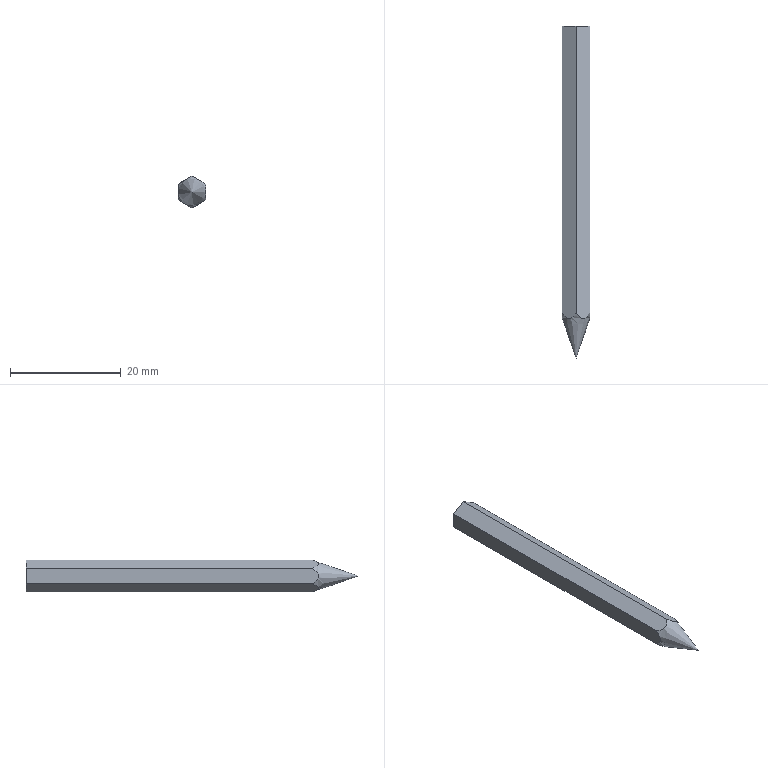Component | NX | 06 | 1 solid | 8 faces | box 5 x 60 x 5.77 mm | volume 1190 mm3 | plane 7 | cone 1
STEP:
#1=CARTESIAN_POINT('',(0.,0.,0.));
#2=DIRECTION('',(0.,0.,1.));
#3=DIRECTION('',(1.,0.,0.));
#4=AXIS2_PLACEMENT_3D('',#1,#2,#3);
#5=CARTESIAN_POINT('',(-22.043,-44.169,-1.443));
#6=VERTEX_POINT('',#5);
#7=CARTESIAN_POINT('',(-22.043,-95.922,-1.443));
#8=VERTEX_POINT('',#7);
#9=CARTESIAN_POINT('',(-22.043,-44.169,-1.443));
#10=DIRECTION('',(0.,-1.,0.));
#11=VECTOR('',#10,1.);
#12=LINE('',#9,#11);
#13=CARTESIAN_POINT('',(-22.043,-44.169,1.443));
#14=DIRECTION('',(-1.,0.,-0.));
#15=DIRECTION('',(0.,0.,-1.));
#16=AXIS2_PLACEMENT_3D('',#13,#14,#15);
#17=PLANE('',#16);
#18=CARTESIAN_POINT('',(2.887,0.));
#19=DIRECTION('',(0.,1.));
#20=VECTOR('',#19,1.);
#21=LINE('',#18,#20);
#22=(GEOMETRIC_REPRESENTATION_CONTEXT(2)PARAMETRIC_REPRESENTATION_CONTEXT()REPRESENTATION_CONTEXT('',''));
#23=DEFINITIONAL_REPRESENTATION('',(#21),#22);
#24=PCURVE('',#17,#23);
#25=CARTESIAN_POINT('',(-22.043,-44.169,-1.443));
#26=DIRECTION('',(-0.5,0.,-0.866));
#27=DIRECTION('',(0.866,0.,-0.5));
#28=AXIS2_PLACEMENT_3D('',#25,#26,#27);
#29=PLANE('',#28);
#30=CARTESIAN_POINT('',(0.,0.));
#31=DIRECTION('',(0.,1.));
#32=VECTOR('',#31,1.);
#33=LINE('',#30,#32);
#34=(GEOMETRIC_REPRESENTATION_CONTEXT(2)PARAMETRIC_REPRESENTATION_CONTEXT()REPRESENTATION_CONTEXT('',''));
#35=DEFINITIONAL_REPRESENTATION('',(#33),#34);
#36=PCURVE('',#29,#35);
#37=SURFACE_CURVE('',#12,(#24,#36),.PCURVE_S1.);
#38=EDGE_CURVE('',#6,#8,#37,.T.);
#39=ORIENTED_EDGE('',*,*,#38,.T.);
#40=CARTESIAN_POINT('',(-22.043,-95.922,1.443));
#41=VERTEX_POINT('',#40);
#42=CARTESIAN_POINT('',(-22.043,-95.922,1.443));
#43=CARTESIAN_POINT('',(-22.043,-96.22,1.235));
#44=CARTESIAN_POINT('',(-22.043,-96.512,1.004));
#45=CARTESIAN_POINT('',(-22.043,-96.738,0.7181));
#46=CARTESIAN_POINT('',(-22.043,-96.826,0.6057));
#47=CARTESIAN_POINT('',(-22.043,-96.905,0.4823));
#48=CARTESIAN_POINT('',(-22.043,-96.957,0.3493));
#49=CARTESIAN_POINT('',(-22.043,-96.996,0.2517));
#50=CARTESIAN_POINT('',(-22.043,-97.02,0.1468));
#51=CARTESIAN_POINT('',(-22.043,-97.026,0.04207));
#52=CARTESIAN_POINT('',(-22.043,-97.031,-0.06307));
#53=CARTESIAN_POINT('',(-22.043,-97.016,-0.1705));
#54=CARTESIAN_POINT('',(-22.043,-96.985,-0.2711));
#55=CARTESIAN_POINT('',(-22.043,-96.944,-0.4017));
#56=CARTESIAN_POINT('',(-22.043,-96.877,-0.5249));
#57=CARTESIAN_POINT('',(-22.043,-96.799,-0.6366));
#58=CARTESIAN_POINT('',(-22.043,-96.614,-0.8978));
#59=CARTESIAN_POINT('',(-22.043,-96.366,-1.113));
#60=CARTESIAN_POINT('',(-22.043,-96.111,-1.305));
#61=CARTESIAN_POINT('',(-22.043,-96.049,-1.353));
#62=CARTESIAN_POINT('',(-22.043,-95.986,-1.399));
#63=CARTESIAN_POINT('',(-22.043,-95.922,-1.443));
#64=B_SPLINE_CURVE_WITH_KNOTS('',3,(#42,#43,#44,#45,#46,#47,#48,#49,#50,#51,#52,#53,#54,#55,#56,#57,#58,#59,#60,#61,#62,#63),.UNSPECIFIED.,.F.,.F.,(4,3,3,3,3,3,3,4),(0.,0.2915,0.4053,0.4887,0.5725,0.6814,0.9377,1.),.UNSPECIFIED.);
#65=CARTESIAN_POINT('',(0.,51.752));
#66=CARTESIAN_POINT('',(0.2087,52.05));
#67=CARTESIAN_POINT('',(0.4395,52.343));
#68=CARTESIAN_POINT('',(0.7253,52.568));
#69=CARTESIAN_POINT('',(0.8376,52.657));
#70=CARTESIAN_POINT('',(0.9611,52.735));
#71=CARTESIAN_POINT('',(1.094,52.788));
#72=CARTESIAN_POINT('',(1.192,52.826));
#73=CARTESIAN_POINT('',(1.297,52.851));
#74=CARTESIAN_POINT('',(1.401,52.856));
#75=CARTESIAN_POINT('',(1.506,52.861));
#76=CARTESIAN_POINT('',(1.614,52.846));
#77=CARTESIAN_POINT('',(1.714,52.815));
#78=CARTESIAN_POINT('',(1.845,52.775));
#79=CARTESIAN_POINT('',(1.968,52.708));
#80=CARTESIAN_POINT('',(2.08,52.629));
#81=CARTESIAN_POINT('',(2.341,52.445));
#82=CARTESIAN_POINT('',(2.556,52.197));
#83=CARTESIAN_POINT('',(2.749,51.942));
#84=CARTESIAN_POINT('',(2.796,51.88));
#85=CARTESIAN_POINT('',(2.842,51.816));
#86=CARTESIAN_POINT('',(2.887,51.752));
#87=B_SPLINE_CURVE_WITH_KNOTS('',3,(#65,#66,#67,#68,#69,#70,#71,#72,#73,#74,#75,#76,#77,#78,#79,#80,#81,#82,#83,#84,#85,#86),.UNSPECIFIED.,.F.,.F.,(4,3,3,3,3,3,3,4),(0.,0.2915,0.4053,0.4887,0.5725,0.6814,0.9377,1.),.UNSPECIFIED.);
#88=(GEOMETRIC_REPRESENTATION_CONTEXT(2)PARAMETRIC_REPRESENTATION_CONTEXT()REPRESENTATION_CONTEXT('',''));
#89=DEFINITIONAL_REPRESENTATION('',(#87),#88);
#90=PCURVE('',#17,#89);
#91=CARTESIAN_POINT('',(-19.543,-104.169,0.00000003));
#92=DIRECTION('',(0.,1.,0.));
#93=DIRECTION('',(0.866,0.,-0.5));
#94=AXIS2_PLACEMENT_3D('',#91,#92,#93);
#95=CONICAL_SURFACE('',#94,0.,0.3367);
#96=CARTESIAN_POINT('',(3.142,8.248));
#97=CARTESIAN_POINT('',(3.137,8.225));
#98=CARTESIAN_POINT('',(3.127,8.178));
#99=CARTESIAN_POINT('',(3.111,8.109));
#100=CARTESIAN_POINT('',(3.095,8.04));
#101=CARTESIAN_POINT('',(3.079,7.972));
#102=CARTESIAN_POINT('',(3.061,7.905));
#103=CARTESIAN_POINT('',(3.044,7.839));
#104=CARTESIAN_POINT('',(3.025,7.775));
#105=CARTESIAN_POINT('',(3.005,7.711));
#106=CARTESIAN_POINT('',(2.985,7.65));
#107=CARTESIAN_POINT('',(2.963,7.59));
#108=CARTESIAN_POINT('',(2.941,7.532));
#109=CARTESIAN_POINT('',(2.918,7.476));
#110=CARTESIAN_POINT('',(2.894,7.422));
#111=CARTESIAN_POINT('',(2.868,7.371));
#112=CARTESIAN_POINT('',(2.841,7.323));
#113=CARTESIAN_POINT('',(2.812,7.279));
#114=CARTESIAN_POINT('',(2.783,7.24));
#115=CARTESIAN_POINT('',(2.752,7.206));
#116=CARTESIAN_POINT('',(2.72,7.179));
#117=CARTESIAN_POINT('',(2.686,7.158));
#118=CARTESIAN_POINT('',(2.652,7.146));
#119=CARTESIAN_POINT('',(2.618,7.141));
#120=CARTESIAN_POINT('',(2.583,7.146));
#121=CARTESIAN_POINT('',(2.549,7.159));
#122=CARTESIAN_POINT('',(2.516,7.179));
#123=CARTESIAN_POINT('',(2.484,7.206));
#124=CARTESIAN_POINT('',(2.453,7.24));
#125=CARTESIAN_POINT('',(2.423,7.279));
#126=CARTESIAN_POINT('',(2.395,7.323));
#127=CARTESIAN_POINT('',(2.368,7.371));
#128=CARTESIAN_POINT('',(2.343,7.422));
#129=CARTESIAN_POINT('',(2.318,7.475));
#130=CARTESIAN_POINT('',(2.295,7.531));
#131=CARTESIAN_POINT('',(2.273,7.589));
#132=CARTESIAN_POINT('',(2.251,7.649));
#133=CARTESIAN_POINT('',(2.231,7.711));
#134=CARTESIAN_POINT('',(2.211,7.775));
#135=CARTESIAN_POINT('',(2.193,7.84));
#136=CARTESIAN_POINT('',(2.175,7.906));
#137=CARTESIAN_POINT('',(2.157,7.973));
#138=CARTESIAN_POINT('',(2.141,8.04));
#139=CARTESIAN_POINT('',(2.125,8.109));
#140=CARTESIAN_POINT('',(2.109,8.178));
#141=CARTESIAN_POINT('',(2.099,8.224));
#142=CARTESIAN_POINT('',(2.094,8.248));
#143=B_SPLINE_CURVE_WITH_KNOTS('',3,(#96,#97,#98,#99,#100,#101,#102,#103,#104,#105,#106,#107,#108,#109,#110,#111,#112,#113,#114,#115,#116,#117,#118,#119,#120,#121,#122,#123,#124,#125,#126,#127,#128,#129,#130,#131,#132,#133,#134,#135,#136,#137,#138,#139,#140,#141,#142),.UNSPECIFIED.,.F.,.F.,(4,1,1,1,1,1,1,1,1,1,1,1,1,1,1,1,1,1,1,1,1,1,1,1,1,1,1,1,1,1,1,1,1,1,1,1,1,1,1,1,1,1,1,1,4),(0.,0.02273,0.04545,0.06818,0.09091,0.1136,0.1364,0.1591,0.1818,0.2045,0.2273,0.25,0.2727,0.2955,0.3182,0.3409,0.3636,0.3864,0.4091,0.4318,0.4545,0.4773,0.5,0.5227,0.5455,0.5682,0.5909,0.6136,0.6364,0.6591,0.6818,0.7045,0.7273,0.75,0.7727,0.7955,0.8182,0.8409,0.8636,0.8864,0.9091,0.9318,0.9545,0.9773,1.),.QUASI_UNIFORM_KNOTS.);
#144=(GEOMETRIC_REPRESENTATION_CONTEXT(2)PARAMETRIC_REPRESENTATION_CONTEXT()REPRESENTATION_CONTEXT('',''));
#145=DEFINITIONAL_REPRESENTATION('',(#143),#144);
#146=PCURVE('',#95,#145);
#147=SURFACE_CURVE('',#64,(#90,#146),.PCURVE_S1.);
#148=EDGE_CURVE('',#41,#8,#147,.T.);
#149=ORIENTED_EDGE('',*,*,#148,.F.);
#150=CARTESIAN_POINT('',(-22.043,-44.169,1.443));
#151=VERTEX_POINT('',#150);
#152=CARTESIAN_POINT('',(-22.043,-44.169,1.443));
#153=DIRECTION('',(0.,-1.,0.));
#154=VECTOR('',#153,1.);
#155=LINE('',#152,#154);
#156=CARTESIAN_POINT('',(0.,0.));
#157=DIRECTION('',(0.,1.));
#158=VECTOR('',#157,1.);
#159=LINE('',#156,#158);
#160=(GEOMETRIC_REPRESENTATION_CONTEXT(2)PARAMETRIC_REPRESENTATION_CONTEXT()REPRESENTATION_CONTEXT('',''));
#161=DEFINITIONAL_REPRESENTATION('',(#159),#160);
#162=PCURVE('',#17,#161);
#163=CARTESIAN_POINT('',(-19.543,-44.169,2.887));
#164=DIRECTION('',(-0.5,0.,0.866));
#165=DIRECTION('',(-0.866,0.,-0.5));
#166=AXIS2_PLACEMENT_3D('',#163,#164,#165);
#167=PLANE('',#166);
#168=CARTESIAN_POINT('',(2.887,0.));
#169=DIRECTION('',(0.,1.));
#170=VECTOR('',#169,1.);
#171=LINE('',#168,#170);
#172=(GEOMETRIC_REPRESENTATION_CONTEXT(2)PARAMETRIC_REPRESENTATION_CONTEXT()REPRESENTATION_CONTEXT('',''));
#173=DEFINITIONAL_REPRESENTATION('',(#171),#172);
#174=PCURVE('',#167,#173);
#175=SURFACE_CURVE('',#155,(#162,#174),.PCURVE_S1.);
#176=EDGE_CURVE('',#151,#41,#175,.T.);
#177=ORIENTED_EDGE('',*,*,#176,.F.);
#178=CARTESIAN_POINT('',(-22.043,-44.169,1.443));
#179=DIRECTION('',(0.,0.,-1.));
#180=VECTOR('',#179,1.);
#181=LINE('',#178,#180);
#182=CARTESIAN_POINT('',(0.,0.));
#183=DIRECTION('',(1.,0.));
#184=VECTOR('',#183,1.);
#185=LINE('',#182,#184);
#186=(GEOMETRIC_REPRESENTATION_CONTEXT(2)PARAMETRIC_REPRESENTATION_CONTEXT()REPRESENTATION_CONTEXT('',''));
#187=DEFINITIONAL_REPRESENTATION('',(#185),#186);
#188=PCURVE('',#17,#187);
#189=CARTESIAN_POINT('',(-19.543,-44.169,0.00000003));
#190=DIRECTION('',(0.,-1.,0.));
#191=DIRECTION('',(0.866,0.,-0.5));
#192=AXIS2_PLACEMENT_3D('',#189,#190,#191);
#193=PLANE('',#192);
#194=CARTESIAN_POINT('',(-2.887,0.));
#195=DIRECTION('',(0.5,-0.866));
#196=VECTOR('',#195,1.);
#197=LINE('',#194,#196);
#198=(GEOMETRIC_REPRESENTATION_CONTEXT(2)PARAMETRIC_REPRESENTATION_CONTEXT()REPRESENTATION_CONTEXT('',''));
#199=DEFINITIONAL_REPRESENTATION('',(#197),#198);
#200=PCURVE('',#193,#199);
#201=SURFACE_CURVE('',#181,(#188,#200),.PCURVE_S1.);
#202=EDGE_CURVE('',#151,#6,#201,.T.);
#203=ORIENTED_EDGE('',*,*,#202,.T.);
#204=EDGE_LOOP('',(#39,#149,#177,#203));
#205=FACE_BOUND('',#204,.T.);
#206=ADVANCED_FACE('',(#205),#17,.T.);
#207=CARTESIAN_POINT('',(-19.543,-44.169,-2.887));
#208=VERTEX_POINT('',#207);
#209=CARTESIAN_POINT('',(-19.543,-95.922,-2.887));
#210=VERTEX_POINT('',#209);
#211=CARTESIAN_POINT('',(-19.543,-44.169,-2.887));
#212=DIRECTION('',(0.,-1.,0.));
#213=VECTOR('',#212,1.);
#214=LINE('',#211,#213);
#215=CARTESIAN_POINT('',(2.887,0.));
#216=DIRECTION('',(0.,1.));
#217=VECTOR('',#216,1.);
#218=LINE('',#215,#217);
#219=(GEOMETRIC_REPRESENTATION_CONTEXT(2)PARAMETRIC_REPRESENTATION_CONTEXT()REPRESENTATION_CONTEXT('',''));
#220=DEFINITIONAL_REPRESENTATION('',(#218),#219);
#221=PCURVE('',#29,#220);
#222=CARTESIAN_POINT('',(-19.543,-44.169,-2.887));
#223=DIRECTION('',(0.5,0.,-0.866));
#224=DIRECTION('',(0.866,0.,0.5));
#225=AXIS2_PLACEMENT_3D('',#222,#223,#224);
#226=PLANE('',#225);
#227=CARTESIAN_POINT('',(0.,0.));
#228=DIRECTION('',(0.,1.));
#229=VECTOR('',#228,1.);
#230=LINE('',#227,#229);
#231=(GEOMETRIC_REPRESENTATION_CONTEXT(2)PARAMETRIC_REPRESENTATION_CONTEXT()REPRESENTATION_CONTEXT('',''));
#232=DEFINITIONAL_REPRESENTATION('',(#230),#231);
#233=PCURVE('',#226,#232);
#234=SURFACE_CURVE('',#214,(#221,#233),.PCURVE_S1.);
#235=EDGE_CURVE('',#208,#210,#234,.T.);
#236=ORIENTED_EDGE('',*,*,#235,.T.);
#237=CARTESIAN_POINT('',(-22.043,-95.922,-1.443));
#238=CARTESIAN_POINT('',(-21.889,-96.175,-1.532));
#239=CARTESIAN_POINT('',(-21.72,-96.425,-1.63));
#240=CARTESIAN_POINT('',(-21.316,-96.848,-1.863));
#241=CARTESIAN_POINT('',(-21.066,-97.027,-2.007));
#242=CARTESIAN_POINT('',(-20.516,-97.026,-2.325));
#243=CARTESIAN_POINT('',(-20.267,-96.846,-2.469));
#244=CARTESIAN_POINT('',(-19.865,-96.424,-2.701));
#245=CARTESIAN_POINT('',(-19.698,-96.178,-2.797));
#246=CARTESIAN_POINT('',(-19.543,-95.922,-2.887));
#247=B_SPLINE_CURVE_WITH_KNOTS('',3,(#237,#238,#239,#240,#241,#242,#243,#244,#245,#246),.UNSPECIFIED.,.F.,.F.,(4,2,2,2,4),(0.,0.25,0.5,0.75,1.),.UNSPECIFIED.);
#248=CARTESIAN_POINT('',(0.,51.752));
#249=CARTESIAN_POINT('',(0.1777,52.006));
#250=CARTESIAN_POINT('',(0.3732,52.256));
#251=CARTESIAN_POINT('',(0.8395,52.679));
#252=CARTESIAN_POINT('',(1.128,52.858));
#253=CARTESIAN_POINT('',(1.763,52.857));
#254=CARTESIAN_POINT('',(2.051,52.676));
#255=CARTESIAN_POINT('',(2.515,52.254));
#256=CARTESIAN_POINT('',(2.707,52.009));
#257=CARTESIAN_POINT('',(2.887,51.752));
#258=B_SPLINE_CURVE_WITH_KNOTS('',3,(#248,#249,#250,#251,#252,#253,#254,#255,#256,#257),.UNSPECIFIED.,.F.,.F.,(4,2,2,2,4),(0.,0.25,0.5,0.75,1.),.UNSPECIFIED.);
#259=(GEOMETRIC_REPRESENTATION_CONTEXT(2)PARAMETRIC_REPRESENTATION_CONTEXT()REPRESENTATION_CONTEXT('',''));
#260=DEFINITIONAL_REPRESENTATION('',(#258),#259);
#261=PCURVE('',#29,#260);
#262=CARTESIAN_POINT('',(2.094,8.248));
#263=CARTESIAN_POINT('',(2.085,8.202));
#264=CARTESIAN_POINT('',(2.065,8.11));
#265=CARTESIAN_POINT('',(2.032,7.974));
#266=CARTESIAN_POINT('',(1.997,7.841));
#267=CARTESIAN_POINT('',(1.959,7.713));
#268=CARTESIAN_POINT('',(1.917,7.59));
#269=CARTESIAN_POINT('',(1.871,7.474));
#270=CARTESIAN_POINT('',(1.82,7.367));
#271=CARTESIAN_POINT('',(1.764,7.275));
#272=CARTESIAN_POINT('',(1.703,7.202));
#273=CARTESIAN_POINT('',(1.639,7.154));
#274=CARTESIAN_POINT('',(1.57,7.137));
#275=CARTESIAN_POINT('',(1.502,7.155));
#276=CARTESIAN_POINT('',(1.437,7.203));
#277=CARTESIAN_POINT('',(1.376,7.277));
#278=CARTESIAN_POINT('',(1.32,7.37));
#279=CARTESIAN_POINT('',(1.269,7.477));
#280=CARTESIAN_POINT('',(1.224,7.592));
#281=CARTESIAN_POINT('',(1.183,7.714));
#282=CARTESIAN_POINT('',(1.145,7.841));
#283=CARTESIAN_POINT('',(1.11,7.973));
#284=CARTESIAN_POINT('',(1.077,8.109));
#285=CARTESIAN_POINT('',(1.057,8.201));
#286=CARTESIAN_POINT('',(1.047,8.248));
#287=B_SPLINE_CURVE_WITH_KNOTS('',3,(#262,#263,#264,#265,#266,#267,#268,#269,#270,#271,#272,#273,#274,#275,#276,#277,#278,#279,#280,#281,#282,#283,#284,#285,#286),.UNSPECIFIED.,.F.,.F.,(4,1,1,1,1,1,1,1,1,1,1,1,1,1,1,1,1,1,1,1,1,1,4),(0.,0.04545,0.09091,0.1364,0.1818,0.2273,0.2727,0.3182,0.3636,0.4091,0.4545,0.5,0.5455,0.5909,0.6364,0.6818,0.7273,0.7727,0.8182,0.8636,0.9091,0.9545,1.),.QUASI_UNIFORM_KNOTS.);
#288=(GEOMETRIC_REPRESENTATION_CONTEXT(2)PARAMETRIC_REPRESENTATION_CONTEXT()REPRESENTATION_CONTEXT('',''));
#289=DEFINITIONAL_REPRESENTATION('',(#287),#288);
#290=PCURVE('',#95,#289);
#291=SURFACE_CURVE('',#247,(#261,#290),.PCURVE_S1.);
#292=EDGE_CURVE('',#8,#210,#291,.T.);
#293=ORIENTED_EDGE('',*,*,#292,.F.);
#294=ORIENTED_EDGE('',*,*,#38,.F.);
#295=CARTESIAN_POINT('',(-22.043,-44.169,-1.443));
#296=DIRECTION('',(0.866,0.,-0.5));
#297=VECTOR('',#296,1.);
#298=LINE('',#295,#297);
#299=CARTESIAN_POINT('',(0.,0.));
#300=DIRECTION('',(1.,0.));
#301=VECTOR('',#300,1.);
#302=LINE('',#299,#301);
#303=(GEOMETRIC_REPRESENTATION_CONTEXT(2)PARAMETRIC_REPRESENTATION_CONTEXT()REPRESENTATION_CONTEXT('',''));
#304=DEFINITIONAL_REPRESENTATION('',(#302),#303);
#305=PCURVE('',#29,#304);
#306=CARTESIAN_POINT('',(-1.443,-2.5));
#307=DIRECTION('',(1.,0.));
#308=VECTOR('',#307,1.);
#309=LINE('',#306,#308);
#310=(GEOMETRIC_REPRESENTATION_CONTEXT(2)PARAMETRIC_REPRESENTATION_CONTEXT()REPRESENTATION_CONTEXT('',''));
#311=DEFINITIONAL_REPRESENTATION('',(#309),#310);
#312=PCURVE('',#193,#311);
#313=SURFACE_CURVE('',#298,(#305,#312),.PCURVE_S1.);
#314=EDGE_CURVE('',#6,#208,#313,.T.);
#315=ORIENTED_EDGE('',*,*,#314,.T.);
#316=EDGE_LOOP('',(#236,#293,#294,#315));
#317=FACE_BOUND('',#316,.T.);
#318=ADVANCED_FACE('',(#317),#29,.T.);
#319=CARTESIAN_POINT('',(-17.043,-44.169,-1.443));
#320=VERTEX_POINT('',#319);
#321=CARTESIAN_POINT('',(-17.043,-95.922,-1.443));
#322=VERTEX_POINT('',#321);
#323=CARTESIAN_POINT('',(-17.043,-44.169,-1.443));
#324=DIRECTION('',(0.,-1.,0.));
#325=VECTOR('',#324,1.);
#326=LINE('',#323,#325);
#327=CARTESIAN_POINT('',(2.887,0.));
#328=DIRECTION('',(0.,1.));
#329=VECTOR('',#328,1.);
#330=LINE('',#327,#329);
#331=(GEOMETRIC_REPRESENTATION_CONTEXT(2)PARAMETRIC_REPRESENTATION_CONTEXT()REPRESENTATION_CONTEXT('',''));
#332=DEFINITIONAL_REPRESENTATION('',(#330),#331);
#333=PCURVE('',#226,#332);
#334=CARTESIAN_POINT('',(-17.043,-44.169,-1.443));
#335=DIRECTION('',(1.,0.,0.));
#336=DIRECTION('',(-0.,0.,1.));
#337=AXIS2_PLACEMENT_3D('',#334,#335,#336);
#338=PLANE('',#337);
#339=CARTESIAN_POINT('',(0.,0.));
#340=DIRECTION('',(0.,1.));
#341=VECTOR('',#340,1.);
#342=LINE('',#339,#341);
#343=(GEOMETRIC_REPRESENTATION_CONTEXT(2)PARAMETRIC_REPRESENTATION_CONTEXT()REPRESENTATION_CONTEXT('',''));
#344=DEFINITIONAL_REPRESENTATION('',(#342),#343);
#345=PCURVE('',#338,#344);
#346=SURFACE_CURVE('',#326,(#333,#345),.PCURVE_S1.);
#347=EDGE_CURVE('',#320,#322,#346,.T.);
#348=ORIENTED_EDGE('',*,*,#347,.T.);
#349=CARTESIAN_POINT('',(-19.543,-95.922,-2.887));
#350=CARTESIAN_POINT('',(-19.362,-96.22,-2.782));
#351=CARTESIAN_POINT('',(-19.162,-96.512,-2.667));
#352=CARTESIAN_POINT('',(-18.915,-96.738,-2.524));
#353=CARTESIAN_POINT('',(-18.817,-96.826,-2.468));
#354=CARTESIAN_POINT('',(-18.711,-96.905,-2.406));
#355=CARTESIAN_POINT('',(-18.595,-96.957,-2.34));
#356=CARTESIAN_POINT('',(-18.511,-96.996,-2.291));
#357=CARTESIAN_POINT('',(-18.42,-97.02,-2.238));
#358=CARTESIAN_POINT('',(-18.329,-97.026,-2.186));
#359=CARTESIAN_POINT('',(-18.238,-97.031,-2.134));
#360=CARTESIAN_POINT('',(-18.145,-97.016,-2.08));
#361=CARTESIAN_POINT('',(-18.058,-96.985,-2.03));
#362=CARTESIAN_POINT('',(-17.945,-96.944,-1.964));
#363=CARTESIAN_POINT('',(-17.838,-96.877,-1.903));
#364=CARTESIAN_POINT('',(-17.742,-96.799,-1.847));
#365=CARTESIAN_POINT('',(-17.515,-96.614,-1.716));
#366=CARTESIAN_POINT('',(-17.329,-96.366,-1.609));
#367=CARTESIAN_POINT('',(-17.162,-96.111,-1.512));
#368=CARTESIAN_POINT('',(-17.121,-96.049,-1.489));
#369=CARTESIAN_POINT('',(-17.082,-95.986,-1.466));
#370=CARTESIAN_POINT('',(-17.043,-95.922,-1.443));
#371=B_SPLINE_CURVE_WITH_KNOTS('',3,(#349,#350,#351,#352,#353,#354,#355,#356,#357,#358,#359,#360,#361,#362,#363,#364,#365,#366,#367,#368,#369,#370),.UNSPECIFIED.,.F.,.F.,(4,3,3,3,3,3,3,4),(0.,0.2915,0.4053,0.4887,0.5725,0.6814,0.9377,1.),.UNSPECIFIED.);
#372=CARTESIAN_POINT('',(0.,51.752));
#373=CARTESIAN_POINT('',(0.2087,52.05));
#374=CARTESIAN_POINT('',(0.4395,52.343));
#375=CARTESIAN_POINT('',(0.7253,52.568));
#376=CARTESIAN_POINT('',(0.8376,52.657));
#377=CARTESIAN_POINT('',(0.9611,52.735));
#378=CARTESIAN_POINT('',(1.094,52.788));
#379=CARTESIAN_POINT('',(1.192,52.826));
#380=CARTESIAN_POINT('',(1.297,52.851));
#381=CARTESIAN_POINT('',(1.401,52.856));
#382=CARTESIAN_POINT('',(1.506,52.861));
#383=CARTESIAN_POINT('',(1.614,52.846));
#384=CARTESIAN_POINT('',(1.714,52.815));
#385=CARTESIAN_POINT('',(1.845,52.775));
#386=CARTESIAN_POINT('',(1.968,52.708));
#387=CARTESIAN_POINT('',(2.08,52.629));
#388=CARTESIAN_POINT('',(2.341,52.445));
#389=CARTESIAN_POINT('',(2.556,52.197));
#390=CARTESIAN_POINT('',(2.749,51.942));
#391=CARTESIAN_POINT('',(2.796,51.88));
#392=CARTESIAN_POINT('',(2.842,51.816));
#393=CARTESIAN_POINT('',(2.887,51.752));
#394=B_SPLINE_CURVE_WITH_KNOTS('',3,(#372,#373,#374,#375,#376,#377,#378,#379,#380,#381,#382,#383,#384,#385,#386,#387,#388,#389,#390,#391,#392,#393),.UNSPECIFIED.,.F.,.F.,(4,3,3,3,3,3,3,4),(0.,0.2915,0.4053,0.4887,0.5725,0.6814,0.9377,1.),.UNSPECIFIED.);
#395=(GEOMETRIC_REPRESENTATION_CONTEXT(2)PARAMETRIC_REPRESENTATION_CONTEXT()REPRESENTATION_CONTEXT('',''));
#396=DEFINITIONAL_REPRESENTATION('',(#394),#395);
#397=PCURVE('',#226,#396);
#398=CARTESIAN_POINT('',(1.047,8.248));
#399=CARTESIAN_POINT('',(1.042,8.225));
#400=CARTESIAN_POINT('',(1.032,8.178));
#401=CARTESIAN_POINT('',(1.017,8.109));
#402=CARTESIAN_POINT('',(1.001,8.04));
#403=CARTESIAN_POINT('',(0.9844,7.972));
#404=CARTESIAN_POINT('',(0.9671,7.905));
#405=CARTESIAN_POINT('',(0.9491,7.839));
#406=CARTESIAN_POINT('',(0.9304,7.775));
#407=CARTESIAN_POINT('',(0.9108,7.711));
#408=CARTESIAN_POINT('',(0.8904,7.65));
#409=CARTESIAN_POINT('',(0.8691,7.59));
#410=CARTESIAN_POINT('',(0.8468,7.532));
#411=CARTESIAN_POINT('',(0.8235,7.476));
#412=CARTESIAN_POINT('',(0.7992,7.422));
#413=CARTESIAN_POINT('',(0.7734,7.371));
#414=CARTESIAN_POINT('',(0.7464,7.323));
#415=CARTESIAN_POINT('',(0.718,7.279));
#416=CARTESIAN_POINT('',(0.6883,7.24));
#417=CARTESIAN_POINT('',(0.6574,7.206));
#418=CARTESIAN_POINT('',(0.6252,7.179));
#419=CARTESIAN_POINT('',(0.5918,7.158));
#420=CARTESIAN_POINT('',(0.5577,7.146));
#421=CARTESIAN_POINT('',(0.5234,7.141));
#422=CARTESIAN_POINT('',(0.489,7.146));
#423=CARTESIAN_POINT('',(0.4549,7.159));
#424=CARTESIAN_POINT('',(0.4216,7.179));
#425=CARTESIAN_POINT('',(0.3896,7.206));
#426=CARTESIAN_POINT('',(0.3586,7.24));
#427=CARTESIAN_POINT('',(0.3289,7.279));
#428=CARTESIAN_POINT('',(0.3005,7.323));
#429=CARTESIAN_POINT('',(0.2735,7.371));
#430=CARTESIAN_POINT('',(0.2481,7.422));
#431=CARTESIAN_POINT('',(0.2237,7.475));
#432=CARTESIAN_POINT('',(0.2004,7.531));
#433=CARTESIAN_POINT('',(0.1782,7.589));
#434=CARTESIAN_POINT('',(0.1569,7.649));
#435=CARTESIAN_POINT('',(0.1365,7.711));
#436=CARTESIAN_POINT('',(0.117,7.775));
#437=CARTESIAN_POINT('',(0.09826,7.84));
#438=CARTESIAN_POINT('',(0.08031,7.906));
#439=CARTESIAN_POINT('',(0.06307,7.973));
#440=CARTESIAN_POINT('',(0.04652,8.04));
#441=CARTESIAN_POINT('',(0.03043,8.109));
#442=CARTESIAN_POINT('',(0.01491,8.178));
#443=CARTESIAN_POINT('',(0.004909,8.224));
#444=CARTESIAN_POINT('',(0.,8.248));
#445=B_SPLINE_CURVE_WITH_KNOTS('',3,(#398,#399,#400,#401,#402,#403,#404,#405,#406,#407,#408,#409,#410,#411,#412,#413,#414,#415,#416,#417,#418,#419,#420,#421,#422,#423,#424,#425,#426,#427,#428,#429,#430,#431,#432,#433,#434,#435,#436,#437,#438,#439,#440,#441,#442,#443,#444),.UNSPECIFIED.,.F.,.F.,(4,1,1,1,1,1,1,1,1,1,1,1,1,1,1,1,1,1,1,1,1,1,1,1,1,1,1,1,1,1,1,1,1,1,1,1,1,1,1,1,1,1,1,1,4),(0.,0.02273,0.04545,0.06818,0.09091,0.1136,0.1364,0.1591,0.1818,0.2045,0.2273,0.25,0.2727,0.2955,0.3182,0.3409,0.3636,0.3864,0.4091,0.4318,0.4545,0.4773,0.5,0.5227,0.5455,0.5682,0.5909,0.6136,0.6364,0.6591,0.6818,0.7045,0.7273,0.75,0.7727,0.7955,0.8182,0.8409,0.8636,0.8864,0.9091,0.9318,0.9545,0.9773,1.),.QUASI_UNIFORM_KNOTS.);
#446=(GEOMETRIC_REPRESENTATION_CONTEXT(2)PARAMETRIC_REPRESENTATION_CONTEXT()REPRESENTATION_CONTEXT('',''));
#447=DEFINITIONAL_REPRESENTATION('',(#445),#446);
#448=PCURVE('',#95,#447);
#449=SURFACE_CURVE('',#371,(#397,#448),.PCURVE_S1.);
#450=EDGE_CURVE('',#210,#322,#449,.T.);
#451=ORIENTED_EDGE('',*,*,#450,.F.);
#452=ORIENTED_EDGE('',*,*,#235,.F.);
#453=CARTESIAN_POINT('',(-19.543,-44.169,-2.887));
#454=DIRECTION('',(0.866,0.,0.5));
#455=VECTOR('',#454,1.);
#456=LINE('',#453,#455);
#457=CARTESIAN_POINT('',(0.,0.));
#458=DIRECTION('',(1.,0.));
#459=VECTOR('',#458,1.);
#460=LINE('',#457,#459);
#461=(GEOMETRIC_REPRESENTATION_CONTEXT(2)PARAMETRIC_REPRESENTATION_CONTEXT()REPRESENTATION_CONTEXT('',''));
#462=DEFINITIONAL_REPRESENTATION('',(#460),#461);
#463=PCURVE('',#226,#462);
#464=CARTESIAN_POINT('',(1.443,-2.5));
#465=DIRECTION('',(0.5,0.866));
#466=VECTOR('',#465,1.);
#467=LINE('',#464,#466);
#468=(GEOMETRIC_REPRESENTATION_CONTEXT(2)PARAMETRIC_REPRESENTATION_CONTEXT()REPRESENTATION_CONTEXT('',''));
#469=DEFINITIONAL_REPRESENTATION('',(#467),#468);
#470=PCURVE('',#193,#469);
#471=SURFACE_CURVE('',#456,(#463,#470),.PCURVE_S1.);
#472=EDGE_CURVE('',#208,#320,#471,.T.);
#473=ORIENTED_EDGE('',*,*,#472,.T.);
#474=EDGE_LOOP('',(#348,#451,#452,#473));
#475=FACE_BOUND('',#474,.T.);
#476=ADVANCED_FACE('',(#475),#226,.T.);
#477=CARTESIAN_POINT('',(-17.043,-44.169,1.443));
#478=VERTEX_POINT('',#477);
#479=CARTESIAN_POINT('',(-17.043,-95.922,1.443));
#480=VERTEX_POINT('',#479);
#481=CARTESIAN_POINT('',(-17.043,-44.169,1.443));
#482=DIRECTION('',(0.,-1.,0.));
#483=VECTOR('',#482,1.);
#484=LINE('',#481,#483);
#485=CARTESIAN_POINT('',(2.887,0.));
#486=DIRECTION('',(0.,1.));
#487=VECTOR('',#486,1.);
#488=LINE('',#485,#487);
#489=(GEOMETRIC_REPRESENTATION_CONTEXT(2)PARAMETRIC_REPRESENTATION_CONTEXT()REPRESENTATION_CONTEXT('',''));
#490=DEFINITIONAL_REPRESENTATION('',(#488),#489);
#491=PCURVE('',#338,#490);
#492=CARTESIAN_POINT('',(-17.043,-44.169,1.443));
#493=DIRECTION('',(0.5,0.,0.866));
#494=DIRECTION('',(0.,-1.,0.));
#495=AXIS2_PLACEMENT_3D('',#492,#493,#494);
#496=PLANE('',#495);
#497=CARTESIAN_POINT('',(0.,0.));
#498=DIRECTION('',(1.,0.));
#499=VECTOR('',#498,1.);
#500=LINE('',#497,#499);
#501=(GEOMETRIC_REPRESENTATION_CONTEXT(2)PARAMETRIC_REPRESENTATION_CONTEXT()REPRESENTATION_CONTEXT('',''));
#502=DEFINITIONAL_REPRESENTATION('',(#500),#501);
#503=PCURVE('',#496,#502);
#504=SURFACE_CURVE('',#484,(#491,#503),.PCURVE_S1.);
#505=EDGE_CURVE('',#478,#480,#504,.T.);
#506=ORIENTED_EDGE('',*,*,#505,.T.);
#507=CARTESIAN_POINT('',(-17.043,-95.922,-1.443));
#508=CARTESIAN_POINT('',(-17.043,-96.22,-1.235));
#509=CARTESIAN_POINT('',(-17.043,-96.512,-1.004));
#510=CARTESIAN_POINT('',(-17.043,-96.738,-0.7181));
#511=CARTESIAN_POINT('',(-17.043,-96.826,-0.6057));
#512=CARTESIAN_POINT('',(-17.043,-96.905,-0.4823));
#513=CARTESIAN_POINT('',(-17.043,-96.957,-0.3493));
#514=CARTESIAN_POINT('',(-17.043,-96.996,-0.2517));
#515=CARTESIAN_POINT('',(-17.043,-97.02,-0.1468));
#516=CARTESIAN_POINT('',(-17.043,-97.026,-0.04207));
#517=CARTESIAN_POINT('',(-17.043,-97.031,0.06307));
#518=CARTESIAN_POINT('',(-17.043,-97.016,0.1705));
#519=CARTESIAN_POINT('',(-17.043,-96.985,0.2711));
#520=CARTESIAN_POINT('',(-17.043,-96.944,0.4017));
#521=CARTESIAN_POINT('',(-17.043,-96.877,0.5249));
#522=CARTESIAN_POINT('',(-17.043,-96.799,0.6366));
#523=CARTESIAN_POINT('',(-17.043,-96.614,0.8978));
#524=CARTESIAN_POINT('',(-17.043,-96.366,1.113));
#525=CARTESIAN_POINT('',(-17.043,-96.111,1.305));
#526=CARTESIAN_POINT('',(-17.043,-96.049,1.353));
#527=CARTESIAN_POINT('',(-17.043,-95.986,1.399));
#528=CARTESIAN_POINT('',(-17.043,-95.922,1.443));
#529=B_SPLINE_CURVE_WITH_KNOTS('',3,(#507,#508,#509,#510,#511,#512,#513,#514,#515,#516,#517,#518,#519,#520,#521,#522,#523,#524,#525,#526,#527,#528),.UNSPECIFIED.,.F.,.F.,(4,3,3,3,3,3,3,4),(0.,0.2915,0.4053,0.4887,0.5725,0.6814,0.9377,1.),.UNSPECIFIED.);
#530=CARTESIAN_POINT('',(0.,51.752));
#531=CARTESIAN_POINT('',(0.2087,52.05));
#532=CARTESIAN_POINT('',(0.4395,52.343));
#533=CARTESIAN_POINT('',(0.7253,52.568));
#534=CARTESIAN_POINT('',(0.8376,52.657));
#535=CARTESIAN_POINT('',(0.9611,52.735));
#536=CARTESIAN_POINT('',(1.094,52.788));
#537=CARTESIAN_POINT('',(1.192,52.826));
#538=CARTESIAN_POINT('',(1.297,52.851));
#539=CARTESIAN_POINT('',(1.401,52.856));
#540=CARTESIAN_POINT('',(1.506,52.861));
#541=CARTESIAN_POINT('',(1.614,52.846));
#542=CARTESIAN_POINT('',(1.714,52.815));
#543=CARTESIAN_POINT('',(1.845,52.775));
#544=CARTESIAN_POINT('',(1.968,52.708));
#545=CARTESIAN_POINT('',(2.08,52.629));
#546=CARTESIAN_POINT('',(2.341,52.445));
#547=CARTESIAN_POINT('',(2.556,52.197));
#548=CARTESIAN_POINT('',(2.749,51.942));
#549=CARTESIAN_POINT('',(2.796,51.88));
#550=CARTESIAN_POINT('',(2.842,51.816));
#551=CARTESIAN_POINT('',(2.887,51.752));
#552=B_SPLINE_CURVE_WITH_KNOTS('',3,(#530,#531,#532,#533,#534,#535,#536,#537,#538,#539,#540,#541,#542,#543,#544,#545,#546,#547,#548,#549,#550,#551),.UNSPECIFIED.,.F.,.F.,(4,3,3,3,3,3,3,4),(0.,0.2915,0.4053,0.4887,0.5725,0.6814,0.9377,1.),.UNSPECIFIED.);
#553=(GEOMETRIC_REPRESENTATION_CONTEXT(2)PARAMETRIC_REPRESENTATION_CONTEXT()REPRESENTATION_CONTEXT('',''));
#554=DEFINITIONAL_REPRESENTATION('',(#552),#553);
#555=PCURVE('',#338,#554);
#556=CARTESIAN_POINT('',(6.283,8.248));
#557=CARTESIAN_POINT('',(6.278,8.225));
#558=CARTESIAN_POINT('',(6.268,8.178));
#559=CARTESIAN_POINT('',(6.253,8.109));
#560=CARTESIAN_POINT('',(6.237,8.04));
#561=CARTESIAN_POINT('',(6.22,7.972));
#562=CARTESIAN_POINT('',(6.203,7.905));
#563=CARTESIAN_POINT('',(6.185,7.839));
#564=CARTESIAN_POINT('',(6.166,7.775));
#565=CARTESIAN_POINT('',(6.147,7.711));
#566=CARTESIAN_POINT('',(6.126,7.65));
#567=CARTESIAN_POINT('',(6.105,7.59));
#568=CARTESIAN_POINT('',(6.083,7.532));
#569=CARTESIAN_POINT('',(6.06,7.476));
#570=CARTESIAN_POINT('',(6.035,7.422));
#571=CARTESIAN_POINT('',(6.009,7.371));
#572=CARTESIAN_POINT('',(5.982,7.323));
#573=CARTESIAN_POINT('',(5.954,7.279));
#574=CARTESIAN_POINT('',(5.924,7.24));
#575=CARTESIAN_POINT('',(5.893,7.206));
#576=CARTESIAN_POINT('',(5.861,7.179));
#577=CARTESIAN_POINT('',(5.828,7.158));
#578=CARTESIAN_POINT('',(5.794,7.146));
#579=CARTESIAN_POINT('',(5.759,7.141));
#580=CARTESIAN_POINT('',(5.725,7.146));
#581=CARTESIAN_POINT('',(5.691,7.159));
#582=CARTESIAN_POINT('',(5.658,7.179));
#583=CARTESIAN_POINT('',(5.626,7.206));
#584=CARTESIAN_POINT('',(5.595,7.24));
#585=CARTESIAN_POINT('',(5.565,7.279));
#586=CARTESIAN_POINT('',(5.537,7.323));
#587=CARTESIAN_POINT('',(5.51,7.371));
#588=CARTESIAN_POINT('',(5.484,7.422));
#589=CARTESIAN_POINT('',(5.46,7.475));
#590=CARTESIAN_POINT('',(5.436,7.531));
#591=CARTESIAN_POINT('',(5.414,7.589));
#592=CARTESIAN_POINT('',(5.393,7.649));
#593=CARTESIAN_POINT('',(5.372,7.711));
#594=CARTESIAN_POINT('',(5.353,7.775));
#595=CARTESIAN_POINT('',(5.334,7.84));
#596=CARTESIAN_POINT('',(5.316,7.906));
#597=CARTESIAN_POINT('',(5.299,7.973));
#598=CARTESIAN_POINT('',(5.283,8.04));
#599=CARTESIAN_POINT('',(5.266,8.109));
#600=CARTESIAN_POINT('',(5.251,8.178));
#601=CARTESIAN_POINT('',(5.241,8.224));
#602=CARTESIAN_POINT('',(5.236,8.248));
#603=B_SPLINE_CURVE_WITH_KNOTS('',3,(#556,#557,#558,#559,#560,#561,#562,#563,#564,#565,#566,#567,#568,#569,#570,#571,#572,#573,#574,#575,#576,#577,#578,#579,#580,#581,#582,#583,#584,#585,#586,#587,#588,#589,#590,#591,#592,#593,#594,#595,#596,#597,#598,#599,#600,#601,#602),.UNSPECIFIED.,.F.,.F.,(4,1,1,1,1,1,1,1,1,1,1,1,1,1,1,1,1,1,1,1,1,1,1,1,1,1,1,1,1,1,1,1,1,1,1,1,1,1,1,1,1,1,1,1,4),(0.,0.02273,0.04545,0.06818,0.09091,0.1136,0.1364,0.1591,0.1818,0.2045,0.2273,0.25,0.2727,0.2955,0.3182,0.3409,0.3636,0.3864,0.4091,0.4318,0.4545,0.4773,0.5,0.5227,0.5455,0.5682,0.5909,0.6136,0.6364,0.6591,0.6818,0.7045,0.7273,0.75,0.7727,0.7955,0.8182,0.8409,0.8636,0.8864,0.9091,0.9318,0.9545,0.9773,1.),.QUASI_UNIFORM_KNOTS.);
#604=(GEOMETRIC_REPRESENTATION_CONTEXT(2)PARAMETRIC_REPRESENTATION_CONTEXT()REPRESENTATION_CONTEXT('',''));
#605=DEFINITIONAL_REPRESENTATION('',(#603),#604);
#606=PCURVE('',#95,#605);
#607=SURFACE_CURVE('',#529,(#555,#606),.PCURVE_S1.);
#608=EDGE_CURVE('',#322,#480,#607,.T.);
#609=ORIENTED_EDGE('',*,*,#608,.F.);
#610=ORIENTED_EDGE('',*,*,#347,.F.);
#611=CARTESIAN_POINT('',(-17.043,-44.169,-1.443));
#612=DIRECTION('',(-0.,0.,1.));
#613=VECTOR('',#612,1.);
#614=LINE('',#611,#613);
#615=CARTESIAN_POINT('',(0.,0.));
#616=DIRECTION('',(1.,0.));
#617=VECTOR('',#616,1.);
#618=LINE('',#615,#617);
#619=(GEOMETRIC_REPRESENTATION_CONTEXT(2)PARAMETRIC_REPRESENTATION_CONTEXT()REPRESENTATION_CONTEXT('',''));
#620=DEFINITIONAL_REPRESENTATION('',(#618),#619);
#621=PCURVE('',#338,#620);
#622=CARTESIAN_POINT('',(2.887,-0.));
#623=DIRECTION('',(-0.5,0.866));
#624=VECTOR('',#623,1.);
#625=LINE('',#622,#624);
#626=(GEOMETRIC_REPRESENTATION_CONTEXT(2)PARAMETRIC_REPRESENTATION_CONTEXT()REPRESENTATION_CONTEXT('',''));
#627=DEFINITIONAL_REPRESENTATION('',(#625),#626);
#628=PCURVE('',#193,#627);
#629=SURFACE_CURVE('',#614,(#621,#628),.PCURVE_S1.);
#630=EDGE_CURVE('',#320,#478,#629,.T.);
#631=ORIENTED_EDGE('',*,*,#630,.T.);
#632=EDGE_LOOP('',(#506,#609,#610,#631));
#633=FACE_BOUND('',#632,.T.);
#634=ADVANCED_FACE('',(#633),#338,.T.);
#635=CARTESIAN_POINT('',(-19.543,-44.169,2.887));
#636=VERTEX_POINT('',#635);
#637=CARTESIAN_POINT('',(-19.543,-95.922,2.887));
#638=VERTEX_POINT('',#637);
#639=CARTESIAN_POINT('',(-19.543,-44.169,2.887));
#640=DIRECTION('',(0.,-1.,0.));
#641=VECTOR('',#640,1.);
#642=LINE('',#639,#641);
#643=CARTESIAN_POINT('',(0.,-2.887));
#644=DIRECTION('',(1.,0.));
#645=VECTOR('',#644,1.);
#646=LINE('',#643,#645);
#647=(GEOMETRIC_REPRESENTATION_CONTEXT(2)PARAMETRIC_REPRESENTATION_CONTEXT()REPRESENTATION_CONTEXT('',''));
#648=DEFINITIONAL_REPRESENTATION('',(#646),#647);
#649=PCURVE('',#496,#648);
#650=CARTESIAN_POINT('',(0.,0.));
#651=DIRECTION('',(0.,1.));
#652=VECTOR('',#651,1.);
#653=LINE('',#650,#652);
#654=(GEOMETRIC_REPRESENTATION_CONTEXT(2)PARAMETRIC_REPRESENTATION_CONTEXT()REPRESENTATION_CONTEXT('',''));
#655=DEFINITIONAL_REPRESENTATION('',(#653),#654);
#656=PCURVE('',#167,#655);
#657=SURFACE_CURVE('',#642,(#649,#656),.PCURVE_S1.);
#658=EDGE_CURVE('',#636,#638,#657,.T.);
#659=ORIENTED_EDGE('',*,*,#658,.T.);
#660=CARTESIAN_POINT('',(-17.043,-95.922,1.443));
#661=CARTESIAN_POINT('',(-17.198,-96.178,1.533));
#662=CARTESIAN_POINT('',(-17.365,-96.424,1.629));
#663=CARTESIAN_POINT('',(-17.767,-96.846,1.861));
#664=CARTESIAN_POINT('',(-18.016,-97.026,2.005));
#665=CARTESIAN_POINT('',(-18.566,-97.027,2.323));
#666=CARTESIAN_POINT('',(-18.816,-96.848,2.467));
#667=CARTESIAN_POINT('',(-19.22,-96.425,2.7));
#668=CARTESIAN_POINT('',(-19.389,-96.175,2.798));
#669=CARTESIAN_POINT('',(-19.543,-95.922,2.887));
#670=B_SPLINE_CURVE_WITH_KNOTS('',3,(#660,#661,#662,#663,#664,#665,#666,#667,#668,#669),.UNSPECIFIED.,.F.,.F.,(4,2,2,2,4),(0.,0.25,0.5,0.75,1.),.UNSPECIFIED.);
#671=CARTESIAN_POINT('',(51.752,0.));
#672=CARTESIAN_POINT('',(52.009,-0.1797));
#673=CARTESIAN_POINT('',(52.254,-0.3721));
#674=CARTESIAN_POINT('',(52.676,-0.836));
#675=CARTESIAN_POINT('',(52.857,-1.124));
#676=CARTESIAN_POINT('',(52.858,-1.759));
#677=CARTESIAN_POINT('',(52.679,-2.047));
#678=CARTESIAN_POINT('',(52.256,-2.514));
#679=CARTESIAN_POINT('',(52.006,-2.709));
#680=CARTESIAN_POINT('',(51.752,-2.887));
#681=B_SPLINE_CURVE_WITH_KNOTS('',3,(#671,#672,#673,#674,#675,#676,#677,#678,#679,#680),.UNSPECIFIED.,.F.,.F.,(4,2,2,2,4),(0.,0.25,0.5,0.75,1.),.UNSPECIFIED.);
#682=(GEOMETRIC_REPRESENTATION_CONTEXT(2)PARAMETRIC_REPRESENTATION_CONTEXT()REPRESENTATION_CONTEXT('',''));
#683=DEFINITIONAL_REPRESENTATION('',(#681),#682);
#684=PCURVE('',#496,#683);
#685=CARTESIAN_POINT('',(5.236,8.248));
#686=CARTESIAN_POINT('',(5.226,8.201));
#687=CARTESIAN_POINT('',(5.206,8.109));
#688=CARTESIAN_POINT('',(5.174,7.973));
#689=CARTESIAN_POINT('',(5.139,7.841));
#690=CARTESIAN_POINT('',(5.101,7.714));
#691=CARTESIAN_POINT('',(5.059,7.592));
#692=CARTESIAN_POINT('',(5.014,7.477));
#693=CARTESIAN_POINT('',(4.963,7.37));
#694=CARTESIAN_POINT('',(4.907,7.277));
#695=CARTESIAN_POINT('',(4.846,7.203));
#696=CARTESIAN_POINT('',(4.782,7.155));
#697=CARTESIAN_POINT('',(4.713,7.137));
#698=CARTESIAN_POINT('',(4.644,7.154));
#699=CARTESIAN_POINT('',(4.58,7.202));
#700=CARTESIAN_POINT('',(4.519,7.275));
#701=CARTESIAN_POINT('',(4.463,7.367));
#702=CARTESIAN_POINT('',(4.412,7.474));
#703=CARTESIAN_POINT('',(4.366,7.59));
#704=CARTESIAN_POINT('',(4.324,7.713));
#705=CARTESIAN_POINT('',(4.286,7.841));
#706=CARTESIAN_POINT('',(4.251,7.974));
#707=CARTESIAN_POINT('',(4.219,8.11));
#708=CARTESIAN_POINT('',(4.198,8.202));
#709=CARTESIAN_POINT('',(4.189,8.248));
#710=B_SPLINE_CURVE_WITH_KNOTS('',3,(#685,#686,#687,#688,#689,#690,#691,#692,#693,#694,#695,#696,#697,#698,#699,#700,#701,#702,#703,#704,#705,#706,#707,#708,#709),.UNSPECIFIED.,.F.,.F.,(4,1,1,1,1,1,1,1,1,1,1,1,1,1,1,1,1,1,1,1,1,1,4),(0.,0.04545,0.09091,0.1364,0.1818,0.2273,0.2727,0.3182,0.3636,0.4091,0.4545,0.5,0.5455,0.5909,0.6364,0.6818,0.7273,0.7727,0.8182,0.8636,0.9091,0.9545,1.),.QUASI_UNIFORM_KNOTS.);
#711=(GEOMETRIC_REPRESENTATION_CONTEXT(2)PARAMETRIC_REPRESENTATION_CONTEXT()REPRESENTATION_CONTEXT('',''));
#712=DEFINITIONAL_REPRESENTATION('',(#710),#711);
#713=PCURVE('',#95,#712);
#714=SURFACE_CURVE('',#670,(#684,#713),.PCURVE_S1.);
#715=EDGE_CURVE('',#480,#638,#714,.T.);
#716=ORIENTED_EDGE('',*,*,#715,.F.);
#717=ORIENTED_EDGE('',*,*,#505,.F.);
#718=CARTESIAN_POINT('',(-17.043,-44.169,1.443));
#719=DIRECTION('',(-0.866,0.,0.5));
#720=VECTOR('',#719,1.);
#721=LINE('',#718,#720);
#722=CARTESIAN_POINT('',(0.,0.));
#723=DIRECTION('',(0.,-1.));
#724=VECTOR('',#723,1.);
#725=LINE('',#722,#724);
#726=(GEOMETRIC_REPRESENTATION_CONTEXT(2)PARAMETRIC_REPRESENTATION_CONTEXT()REPRESENTATION_CONTEXT('',''));
#727=DEFINITIONAL_REPRESENTATION('',(#725),#726);
#728=PCURVE('',#496,#727);
#729=CARTESIAN_POINT('',(1.443,2.5));
#730=DIRECTION('',(-1.,0.));
#731=VECTOR('',#730,1.);
#732=LINE('',#729,#731);
#733=(GEOMETRIC_REPRESENTATION_CONTEXT(2)PARAMETRIC_REPRESENTATION_CONTEXT()REPRESENTATION_CONTEXT('',''));
#734=DEFINITIONAL_REPRESENTATION('',(#732),#733);
#735=PCURVE('',#193,#734);
#736=SURFACE_CURVE('',#721,(#728,#735),.PCURVE_S1.);
#737=EDGE_CURVE('',#478,#636,#736,.T.);
#738=ORIENTED_EDGE('',*,*,#737,.T.);
#739=EDGE_LOOP('',(#659,#716,#717,#738));
#740=FACE_BOUND('',#739,.T.);
#741=ADVANCED_FACE('',(#740),#496,.T.);
#742=ORIENTED_EDGE('',*,*,#176,.T.);
#743=CARTESIAN_POINT('',(-19.543,-95.922,2.887));
#744=CARTESIAN_POINT('',(-19.724,-96.22,2.782));
#745=CARTESIAN_POINT('',(-19.924,-96.512,2.667));
#746=CARTESIAN_POINT('',(-20.171,-96.738,2.524));
#747=CARTESIAN_POINT('',(-20.268,-96.826,2.468));
#748=CARTESIAN_POINT('',(-20.375,-96.905,2.406));
#749=CARTESIAN_POINT('',(-20.49,-96.957,2.34));
#750=CARTESIAN_POINT('',(-20.575,-96.996,2.291));
#751=CARTESIAN_POINT('',(-20.666,-97.02,2.238));
#752=CARTESIAN_POINT('',(-20.756,-97.026,2.186));
#753=CARTESIAN_POINT('',(-20.848,-97.031,2.134));
#754=CARTESIAN_POINT('',(-20.941,-97.016,2.08));
#755=CARTESIAN_POINT('',(-21.028,-96.985,2.03));
#756=CARTESIAN_POINT('',(-21.141,-96.944,1.964));
#757=CARTESIAN_POINT('',(-21.247,-96.877,1.903));
#758=CARTESIAN_POINT('',(-21.344,-96.799,1.847));
#759=CARTESIAN_POINT('',(-21.57,-96.614,1.716));
#760=CARTESIAN_POINT('',(-21.756,-96.366,1.609));
#761=CARTESIAN_POINT('',(-21.923,-96.111,1.512));
#762=CARTESIAN_POINT('',(-21.964,-96.049,1.489));
#763=CARTESIAN_POINT('',(-22.004,-95.986,1.466));
#764=CARTESIAN_POINT('',(-22.043,-95.922,1.443));
#765=B_SPLINE_CURVE_WITH_KNOTS('',3,(#743,#744,#745,#746,#747,#748,#749,#750,#751,#752,#753,#754,#755,#756,#757,#758,#759,#760,#761,#762,#763,#764),.UNSPECIFIED.,.F.,.F.,(4,3,3,3,3,3,3,4),(0.,0.2915,0.4053,0.4887,0.5725,0.6814,0.9377,1.),.UNSPECIFIED.);
#766=CARTESIAN_POINT('',(0.,51.752));
#767=CARTESIAN_POINT('',(0.2087,52.05));
#768=CARTESIAN_POINT('',(0.4395,52.343));
#769=CARTESIAN_POINT('',(0.7253,52.568));
#770=CARTESIAN_POINT('',(0.8376,52.657));
#771=CARTESIAN_POINT('',(0.9611,52.735));
#772=CARTESIAN_POINT('',(1.094,52.788));
#773=CARTESIAN_POINT('',(1.192,52.826));
#774=CARTESIAN_POINT('',(1.297,52.851));
#775=CARTESIAN_POINT('',(1.401,52.856));
#776=CARTESIAN_POINT('',(1.506,52.861));
#777=CARTESIAN_POINT('',(1.614,52.846));
#778=CARTESIAN_POINT('',(1.714,52.815));
#779=CARTESIAN_POINT('',(1.845,52.775));
#780=CARTESIAN_POINT('',(1.968,52.708));
#781=CARTESIAN_POINT('',(2.08,52.629));
#782=CARTESIAN_POINT('',(2.341,52.445));
#783=CARTESIAN_POINT('',(2.556,52.197));
#784=CARTESIAN_POINT('',(2.749,51.942));
#785=CARTESIAN_POINT('',(2.796,51.88));
#786=CARTESIAN_POINT('',(2.842,51.816));
#787=CARTESIAN_POINT('',(2.887,51.752));
#788=B_SPLINE_CURVE_WITH_KNOTS('',3,(#766,#767,#768,#769,#770,#771,#772,#773,#774,#775,#776,#777,#778,#779,#780,#781,#782,#783,#784,#785,#786,#787),.UNSPECIFIED.,.F.,.F.,(4,3,3,3,3,3,3,4),(0.,0.2915,0.4053,0.4887,0.5725,0.6814,0.9377,1.),.UNSPECIFIED.);
#789=(GEOMETRIC_REPRESENTATION_CONTEXT(2)PARAMETRIC_REPRESENTATION_CONTEXT()REPRESENTATION_CONTEXT('',''));
#790=DEFINITIONAL_REPRESENTATION('',(#788),#789);
#791=PCURVE('',#167,#790);
#792=CARTESIAN_POINT('',(4.189,8.248));
#793=CARTESIAN_POINT('',(4.184,8.225));
#794=CARTESIAN_POINT('',(4.174,8.178));
#795=CARTESIAN_POINT('',(4.159,8.109));
#796=CARTESIAN_POINT('',(4.143,8.04));
#797=CARTESIAN_POINT('',(4.126,7.972));
#798=CARTESIAN_POINT('',(4.109,7.905));
#799=CARTESIAN_POINT('',(4.091,7.839));
#800=CARTESIAN_POINT('',(4.072,7.775));
#801=CARTESIAN_POINT('',(4.052,7.711));
#802=CARTESIAN_POINT('',(4.032,7.65));
#803=CARTESIAN_POINT('',(4.011,7.59));
#804=CARTESIAN_POINT('',(3.988,7.532));
#805=CARTESIAN_POINT('',(3.965,7.476));
#806=CARTESIAN_POINT('',(3.941,7.422));
#807=CARTESIAN_POINT('',(3.915,7.371));
#808=CARTESIAN_POINT('',(3.888,7.323));
#809=CARTESIAN_POINT('',(3.86,7.279));
#810=CARTESIAN_POINT('',(3.83,7.24));
#811=CARTESIAN_POINT('',(3.799,7.206));
#812=CARTESIAN_POINT('',(3.767,7.179));
#813=CARTESIAN_POINT('',(3.733,7.158));
#814=CARTESIAN_POINT('',(3.699,7.146));
#815=CARTESIAN_POINT('',(3.665,7.141));
#816=CARTESIAN_POINT('',(3.631,7.146));
#817=CARTESIAN_POINT('',(3.596,7.159));
#818=CARTESIAN_POINT('',(3.563,7.179));
#819=CARTESIAN_POINT('',(3.531,7.206));
#820=CARTESIAN_POINT('',(3.5,7.24));
#821=CARTESIAN_POINT('',(3.471,7.279));
#822=CARTESIAN_POINT('',(3.442,7.323));
#823=CARTESIAN_POINT('',(3.415,7.371));
#824=CARTESIAN_POINT('',(3.39,7.422));
#825=CARTESIAN_POINT('',(3.365,7.475));
#826=CARTESIAN_POINT('',(3.342,7.531));
#827=CARTESIAN_POINT('',(3.32,7.589));
#828=CARTESIAN_POINT('',(3.298,7.649));
#829=CARTESIAN_POINT('',(3.278,7.711));
#830=CARTESIAN_POINT('',(3.259,7.775));
#831=CARTESIAN_POINT('',(3.24,7.84));
#832=CARTESIAN_POINT('',(3.222,7.906));
#833=CARTESIAN_POINT('',(3.205,7.973));
#834=CARTESIAN_POINT('',(3.188,8.04));
#835=CARTESIAN_POINT('',(3.172,8.109));
#836=CARTESIAN_POINT('',(3.156,8.178));
#837=CARTESIAN_POINT('',(3.147,8.224));
#838=CARTESIAN_POINT('',(3.142,8.248));
#839=B_SPLINE_CURVE_WITH_KNOTS('',3,(#792,#793,#794,#795,#796,#797,#798,#799,#800,#801,#802,#803,#804,#805,#806,#807,#808,#809,#810,#811,#812,#813,#814,#815,#816,#817,#818,#819,#820,#821,#822,#823,#824,#825,#826,#827,#828,#829,#830,#831,#832,#833,#834,#835,#836,#837,#838),.UNSPECIFIED.,.F.,.F.,(4,1,1,1,1,1,1,1,1,1,1,1,1,1,1,1,1,1,1,1,1,1,1,1,1,1,1,1,1,1,1,1,1,1,1,1,1,1,1,1,1,1,1,1,4),(0.,0.02273,0.04545,0.06818,0.09091,0.1136,0.1364,0.1591,0.1818,0.2045,0.2273,0.25,0.2727,0.2955,0.3182,0.3409,0.3636,0.3864,0.4091,0.4318,0.4545,0.4773,0.5,0.5227,0.5455,0.5682,0.5909,0.6136,0.6364,0.6591,0.6818,0.7045,0.7273,0.75,0.7727,0.7955,0.8182,0.8409,0.8636,0.8864,0.9091,0.9318,0.9545,0.9773,1.),.QUASI_UNIFORM_KNOTS.);
#840=(GEOMETRIC_REPRESENTATION_CONTEXT(2)PARAMETRIC_REPRESENTATION_CONTEXT()REPRESENTATION_CONTEXT('',''));
#841=DEFINITIONAL_REPRESENTATION('',(#839),#840);
#842=PCURVE('',#95,#841);
#843=SURFACE_CURVE('',#765,(#791,#842),.PCURVE_S1.);
#844=EDGE_CURVE('',#638,#41,#843,.T.);
#845=ORIENTED_EDGE('',*,*,#844,.F.);
#846=ORIENTED_EDGE('',*,*,#658,.F.);
#847=CARTESIAN_POINT('',(-19.543,-44.169,2.887));
#848=DIRECTION('',(-0.866,0.,-0.5));
#849=VECTOR('',#848,1.);
#850=LINE('',#847,#849);
#851=CARTESIAN_POINT('',(0.,0.));
#852=DIRECTION('',(1.,0.));
#853=VECTOR('',#852,1.);
#854=LINE('',#851,#853);
#855=(GEOMETRIC_REPRESENTATION_CONTEXT(2)PARAMETRIC_REPRESENTATION_CONTEXT()REPRESENTATION_CONTEXT('',''));
#856=DEFINITIONAL_REPRESENTATION('',(#854),#855);
#857=PCURVE('',#167,#856);
#858=CARTESIAN_POINT('',(-1.443,2.5));
#859=DIRECTION('',(-0.5,-0.866));
#860=VECTOR('',#859,1.);
#861=LINE('',#858,#860);
#862=(GEOMETRIC_REPRESENTATION_CONTEXT(2)PARAMETRIC_REPRESENTATION_CONTEXT()REPRESENTATION_CONTEXT('',''));
#863=DEFINITIONAL_REPRESENTATION('',(#861),#862);
#864=PCURVE('',#193,#863);
#865=SURFACE_CURVE('',#850,(#857,#864),.PCURVE_S1.);
#866=EDGE_CURVE('',#636,#151,#865,.T.);
#867=ORIENTED_EDGE('',*,*,#866,.T.);
#868=EDGE_LOOP('',(#742,#845,#846,#867));
#869=FACE_BOUND('',#868,.T.);
#870=ADVANCED_FACE('',(#869),#167,.T.);
#871=ORIENTED_EDGE('',*,*,#202,.F.);
#872=ORIENTED_EDGE('',*,*,#866,.F.);
#873=ORIENTED_EDGE('',*,*,#737,.F.);
#874=ORIENTED_EDGE('',*,*,#630,.F.);
#875=ORIENTED_EDGE('',*,*,#472,.F.);
#876=ORIENTED_EDGE('',*,*,#314,.F.);
#877=EDGE_LOOP('',(#871,#872,#873,#874,#875,#876));
#878=FACE_BOUND('',#877,.T.);
#879=ADVANCED_FACE('',(#878),#193,.F.);
#880=CARTESIAN_POINT('',(-19.543,-104.169,0.00000003));
#881=VERTEX_POINT('',#880);
#882=CARTESIAN_POINT('',(-19.543,-104.169,0.00000003));
#883=CARTESIAN_POINT('',(-17.043,-95.922,-1.443));
#884=B_SPLINE_CURVE_WITH_KNOTS('',1,(#882,#883),.UNSPECIFIED.,.F.,.F.,(2,2),(0.,8.738),.PIECEWISE_BEZIER_KNOTS.);
#885=CARTESIAN_POINT('',(6.283,0.));
#886=DIRECTION('',(0.,1.));
#887=VECTOR('',#886,1.);
#888=LINE('',#885,#887);
#889=(GEOMETRIC_REPRESENTATION_CONTEXT(2)PARAMETRIC_REPRESENTATION_CONTEXT()REPRESENTATION_CONTEXT('',''));
#890=DEFINITIONAL_REPRESENTATION('',(#888),#889);
#891=PCURVE('',#95,#890);
#892=CARTESIAN_POINT('',(0.,0.));
#893=DIRECTION('',(0.,1.));
#894=VECTOR('',#893,1.);
#895=LINE('',#892,#894);
#896=(GEOMETRIC_REPRESENTATION_CONTEXT(2)PARAMETRIC_REPRESENTATION_CONTEXT()REPRESENTATION_CONTEXT('',''));
#897=DEFINITIONAL_REPRESENTATION('',(#895),#896);
#898=PCURVE('',#95,#897);
#899=SEAM_CURVE('',#884,(#891,#898),.PCURVE_S1.);
#900=EDGE_CURVE('',#881,#322,#899,.T.);
#901=ORIENTED_EDGE('',*,*,#900,.T.);
#902=ORIENTED_EDGE('',*,*,#608,.T.);
#903=ORIENTED_EDGE('',*,*,#715,.T.);
#904=ORIENTED_EDGE('',*,*,#844,.T.);
#905=ORIENTED_EDGE('',*,*,#148,.T.);
#906=ORIENTED_EDGE('',*,*,#292,.T.);
#907=ORIENTED_EDGE('',*,*,#450,.T.);
#908=ORIENTED_EDGE('',*,*,#900,.F.);
#909=EDGE_LOOP('',(#901,#902,#903,#904,#905,#906,#907,#908));
#910=FACE_BOUND('',#909,.T.);
#911=ADVANCED_FACE('',(#910),#95,.T.);
#912=CLOSED_SHELL('',(#206,#318,#476,#634,#741,#870,#879,#911));
#913=MANIFOLD_SOLID_BREP('',#912);
#914=(LENGTH_UNIT()NAMED_UNIT(*)SI_UNIT(.MILLI.,.METRE.));
#915=UNCERTAINTY_MEASURE_WITH_UNIT(LENGTH_MEASURE(0.0002),#914,'','');
#916=(NAMED_UNIT(*)PLANE_ANGLE_UNIT()SI_UNIT($,.RADIAN.));
#917=(NAMED_UNIT(*)SI_UNIT($,.STERADIAN.)SOLID_ANGLE_UNIT());
#918=(GEOMETRIC_REPRESENTATION_CONTEXT(3)GLOBAL_UNCERTAINTY_ASSIGNED_CONTEXT((#915))GLOBAL_UNIT_ASSIGNED_CONTEXT((#914,#916,#917))REPRESENTATION_CONTEXT('',''));
#919=ADVANCED_BREP_SHAPE_REPRESENTATION('',(#4,#913),#918);